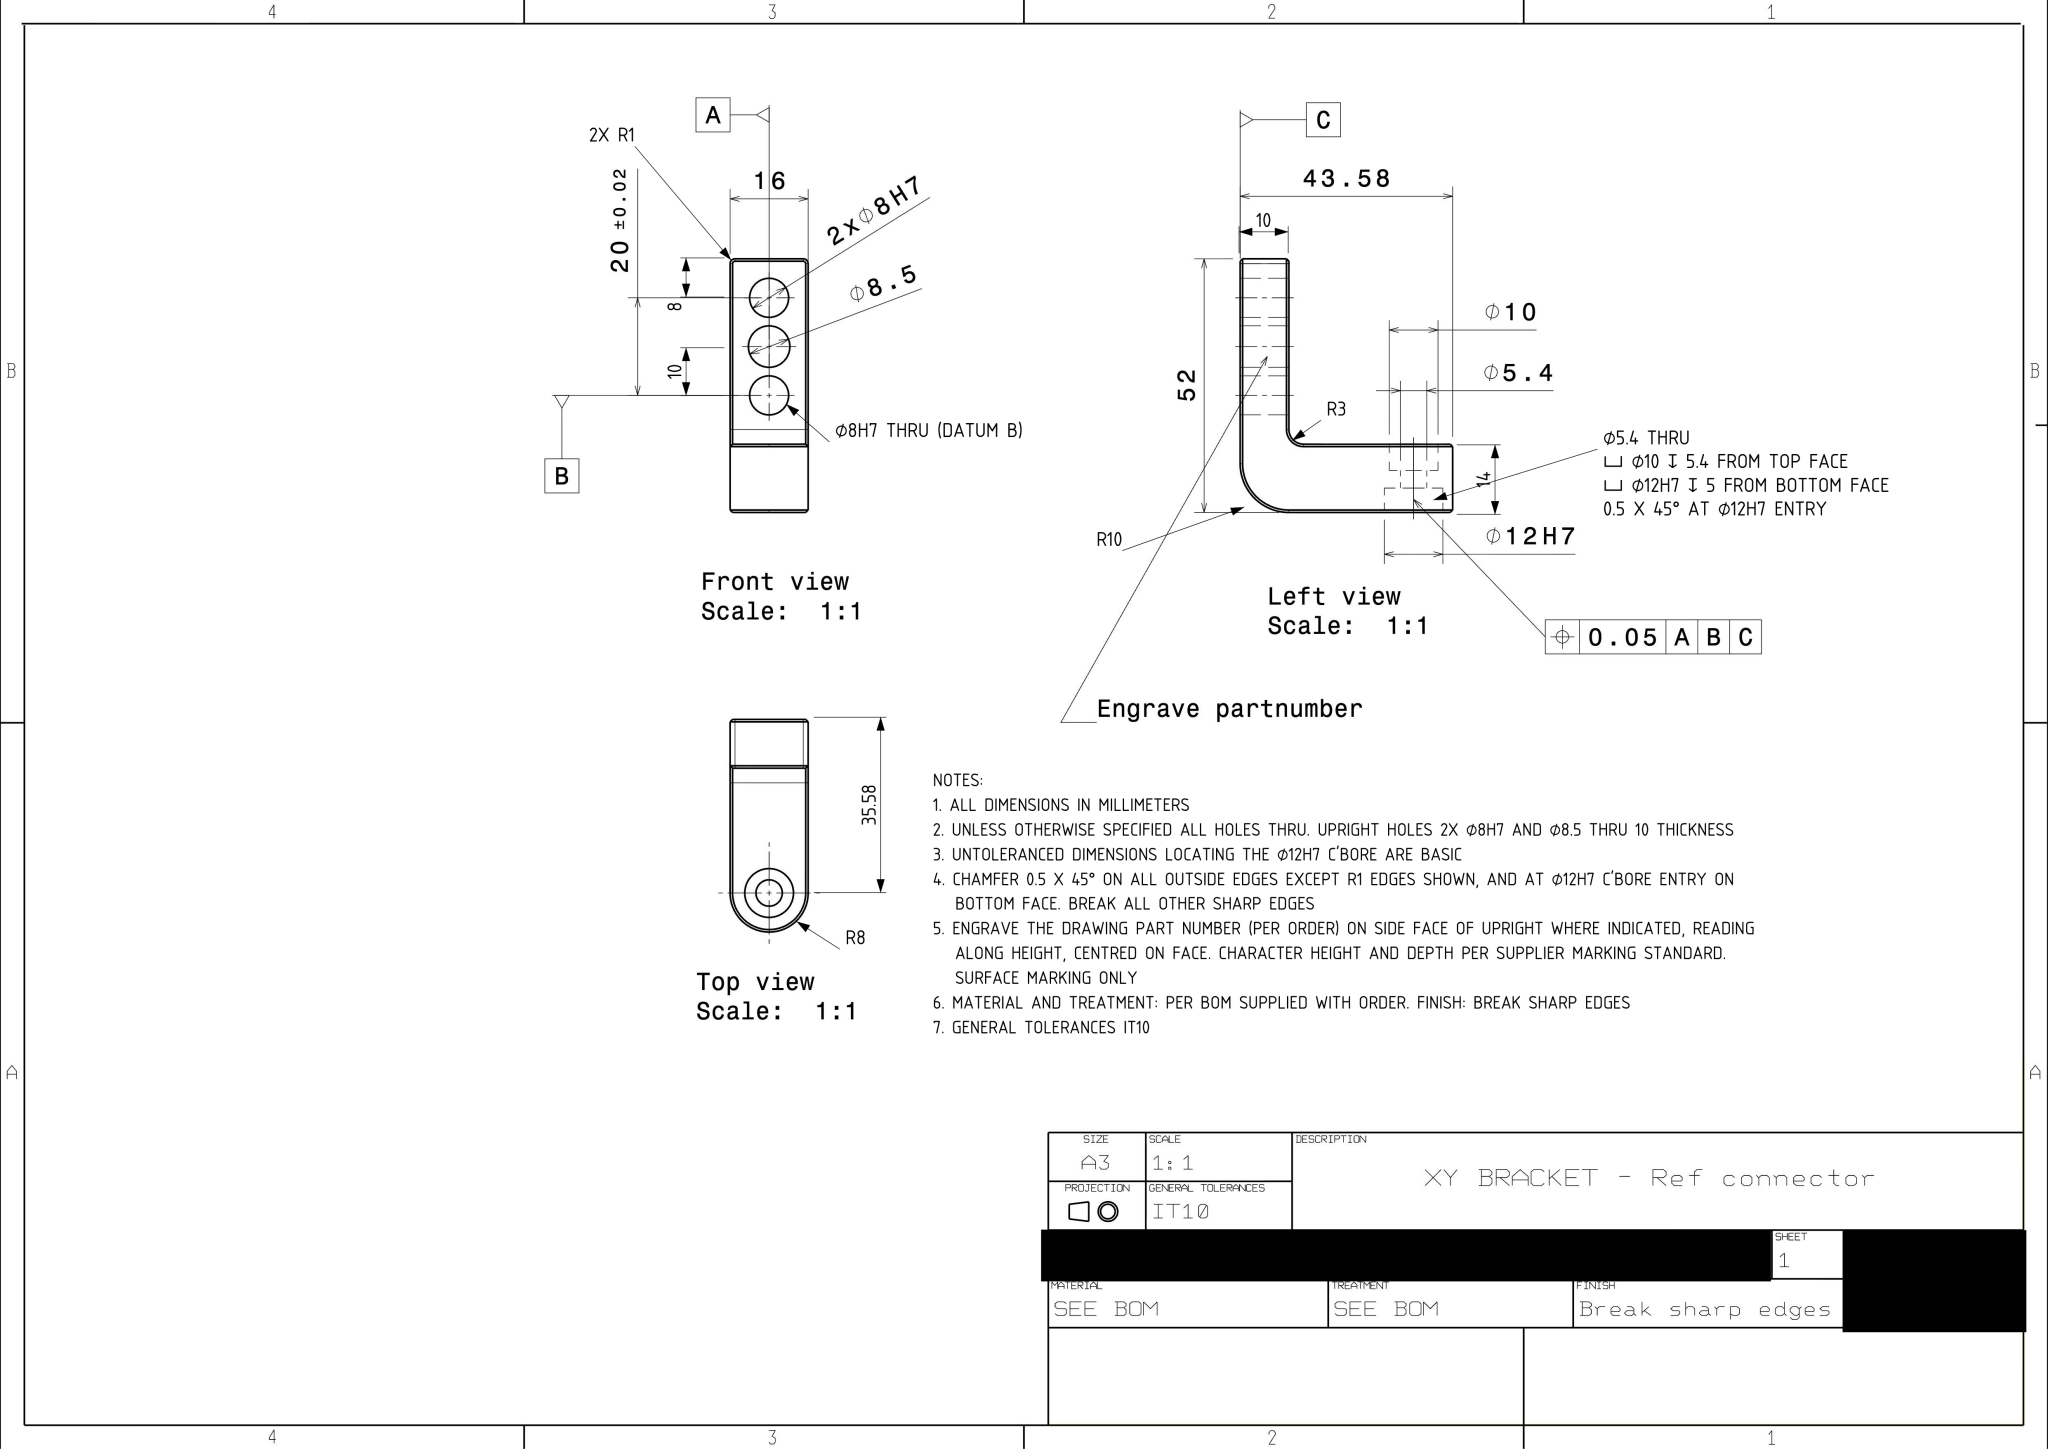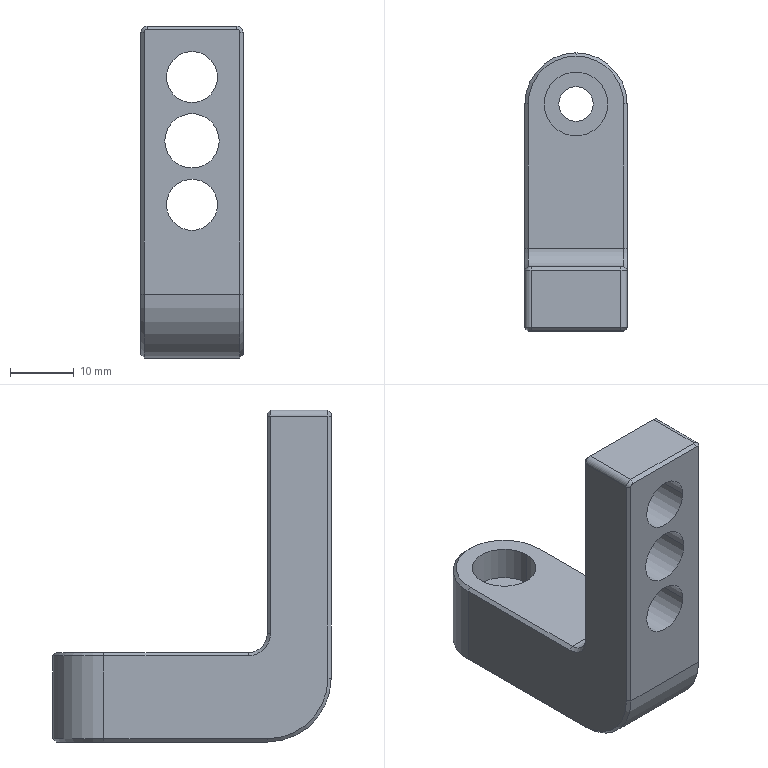Part | NX | mm | 1 solid | 51 faces | box 16 x 43.58 x 52 mm | volume 12445 mm3 | plane 19 | cylinder 18 | cone 14 | commonest cylinder face diameters 8 x4 8.5 x2 2 x2 16 x2 5.4 x2 10 x2 12 x2 20 x1